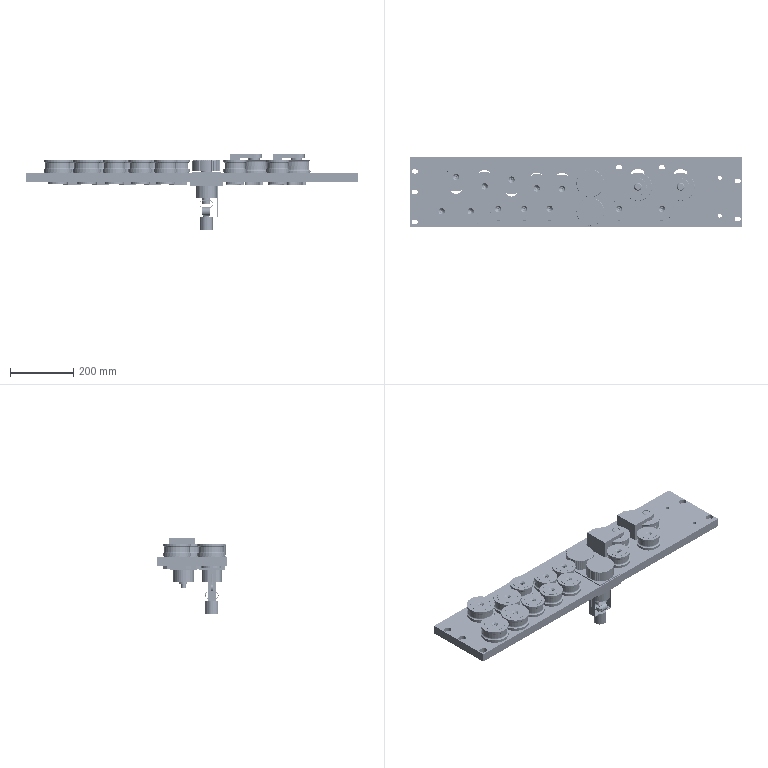Assembly | SolidWorks | mm | 86 component files | 278 solids | 5962 faces | box 1050 x 220 x 237.51 mm | volume 10326215 mm3 | cylinder 1953 | plane 1541 | sphere 1504 | cone 570 | torus 394 | commonest cylinder face diameters 34.9 x282 37.1 x282 8.5 x124 88 x88 86 x86 11 x74 45 x67 55 x64
Bill of materials:
12ACoupling | 1 |  | Two thin-walled stadium (obround) loops arranged at right angles to each other and touching at one point. Each loop holds a cylindrical collar with a central through bore and a small radial hole with a recessed socket feature on its side.
12AEncoder | 1 |  | Solid cylindrical body. A smaller coaxial cylindrical boss sits on one end face, and a thin shaft sticks out of the boss. Three small holes are spaced evenly around the end face.
12AEncoderBracket | 1 | Q235 | Formed sheet-style U-shaped bracket. The flat base has a circular lobe with a large central hole and three small holes around it. Two vertical side walls each have a long vertical slot. Each wall ends in an outward-bent tab with one hole and rounded corners.
12A6005RZBearing | 6 |  | Flat annular ring with a plain cylindrical outer surface and a smooth through-bore. The end face has concentric bands: an outer rim, a wide middle annular face, and a narrow inner ring band near the bore, separated by shallow circular grooves/steps. Overall it looks like a shielded deep-groove ball bearing (outer ring, shield, inner ring), but this is only inferred from shape.
12A6006RZBearing | 2 |  | Annular ring with a rectangular cross-section and rounded edges. The face has shallow concentric step or groove rings between the inner and outer diameters.
12AEncoderAxis | 2 |  | Axisymmetric pin with a large cylindrical head ridged around its edge. Below the head is a stepped shaft that gets narrower in stages. Near the lower end there is a narrow groove and a small end pilot.
12AEncoderAxisFrontBaffle | 2 | Q235 | Thin square plate with a central round through hole. Below the plate is a slightly smaller block with a rounded-square outline.
12AEncoderAxisRearBaffle | 2 | Q235 | Flanged cylindrical housing. A rectangular flange plate has four larger corner holes, two small holes on the short-side centerlines, and a large central through bore. A cylindrical body extends below the plate and a short stepped spigot rises above it.
12AFlatSlotLargeStraighteningWheel | 4 | GCr15 | Spool-shaped wheel with two end flanges and a concave circumferential groove between them. It has a central through bore and a shallow annular groove on the end face.
12ALargeStraighteningWheelAxis | 4 | Q235 | Stepped axisymmetric part. A wide thin flange disc has raised concentric step rings on top. An upper cylinder with a small central hole rises from it, and a larger lower cylinder with chamfered ends sits below.
12ALargeStraighteningWheelCover | 4 | 45 | Thin flat disc with a central countersunk through hole. A shallow stepped boss with a chamfered edge sits on the underside.
12AFixedLargeStraighteningWheelBaffle | 7 | Q235 | Plain flat circular disc with a small central through hole.
12AFlatSlotSmallStraighteningWheel | 8 | GCr15 | Spool-shaped wheel with two end flanges and a concave radiused groove between them. It has a central through bore and an annular groove on the end face. It is proportionally taller, with a relatively larger bore than the similar spool part.
12ASmallStraighteningWheelAxis | 8 | 45 | Stepped, mostly revolved body: a small cylindrical boss on top with a small central hole, a raised annular step, a thin wide flange, and a larger lower cylindrical body with one flat side.
12ASmallStraighteningWheelCover | 8 | 45 | Thin flat circular disc with a central countersunk through hole, plus a shallow stepped boss on the underside.
12A6006DeepGrooveBallBearing | 4 | GCr4 | Ball-bearing-like geometry: concentric outer and inner rings with a ring of spherical balls between them. No shield or cage is visible.
12AInnerSideWheel | 2 | Cr12MoV | Short annular ring with a central through bore and a thin outward flange at its base, joined to the ring wall by a fillet.
12AInnerSideWheelAxis | 2 | 45 | Stepped, mostly revolved body: a solid small cylindrical boss on top, a raised annular step, two flange tiers, and a larger lower cylindrical body with one flat side.
12AOuterSideWheel | 2 | Cr12MoV | Flanged cylindrical sleeve: a short tube with a thin outward flange at one end and a stepped internal bore.
12AOuterSideWheelPlate | 2 | Q235 | Flat plate of uniform thickness: two straight edges meeting at a corner, an angled edge, and a rounded lobe at one end with a single round through hole. There is a small rectangular notch in one edge.
12AOuterSideWheelSeat | 2 | Q235 | T-shaped block: a rectangular upper block with a narrow raised rib running along its top, and a narrower lower extension with a rounded end.
12AOuterSideWheelSmallAxis | 2 | 45 | Solid stepped cylindrical plug: a chamfered top cylinder, a wider collar or flange, and a main cylindrical body with a circumferential groove near the lower end.
12ASlidingPlateWheelCover | 4 | Q235 | Flat rectangular plate with rounded corners, a concave circular-arc cutout along one short edge, and two round through holes in line on the centerline.
12ASlidingStraighteningWheelRetainingPlate | 5 | Q235 | Flat rectangular plate with all four corners chamfered (elongated octagon outline) and two round through holes on the centerline.
12AStraighteningPlate | 1 | Q235 | Long, thin rectangular panel plate with many cutouts in two rows: rounded or D-shaped oblong openings, two square openings, two narrow slots, and small holes and slots near both ends.
Mates:
1. coincident | 12AStraighteningPlate-1 face at (-449.402, 230.038, 14.25) dir (0, 0, 1) | 12AFixedFlatGrooveLargeWheel-EngravingAndMillingAxis-2/12ALargeStraighteningWheelAxis-1 face at (-257.402, 101.538, 14.25) dir (0, 0, -1)
2. coincident | 12AStraighteningPlate-1 face at (-449.402, 230.038, 14.25) dir (0, 0, 1) | 12AFixedFlatGrooveLargeWheel-EngravingAndMillingAxis-3/12ALargeStraighteningWheelAxis-1 face at (-349.402, 101.538, 14.25) dir (0, 0, -1)
3. coincident | 12AStraighteningPlate-1 face at (-363.544, 76.538, -14.25) dir (0, -1, 0) | 12AFixedFlatGrooveLargeWheel-EngravingAndMillingAxis-3/12ALargeStraighteningWheelAxis-1 face at (-335.259, 76.538, 42.973) dir (0, 1, 0)
4. concentric | 12AStraighteningPlate-1 face at (-349.402, 59.038, -14.25) dir (0, 0, 1) r 22.5 | 12AFixedFlatGrooveLargeWheel-EngravingAndMillingAxis-3/12ALargeStraighteningWheelAxis-1 face at (-349.402, 59.038, -14.25) dir (0, 0, -1) r 22.5
5. coincident | 12AStraighteningPlate-1 face at (-271.544, 76.538, -14.25) dir (0, -1, 0) | 12AFixedFlatGrooveLargeWheel-EngravingAndMillingAxis-2/12ALargeStraighteningWheelAxis-1 face at (-243.259, 76.538, 42.973) dir (0, 1, 0)
6. concentric | 12AStraighteningPlate-1 face at (-257.402, 59.038, -14.25) dir (0, 0, 1) r 22.5 | 12AFixedFlatGrooveLargeWheel-EngravingAndMillingAxis-2/12ALargeStraighteningWheelAxis-1 face at (-257.402, 59.038, -14.25) dir (0, 0, -1) r 22.5
7. coincident | 12AStraighteningPlate-1 face at (-449.402, 230.038, 14.25) dir (0, 0, 1) | 12AFlatGrooveSmallWheel-MillingAxis-5/12ASmallStraighteningWheelAxis-1 face at (346.598, 101.038, 14.25) dir (0, 0, -1)
8. coincident | 12AStraighteningPlate-1 face at (-449.402, 230.038, 14.25) dir (0, 0, 1) | 12AFlatGrooveSmallWheel-MillingAxis-4/12ASmallStraighteningWheelAxis-1 face at (211.598, 101.038, 14.25) dir (0, 0, -1)
9. coincident | 12AStraighteningPlate-1 face at (-449.402, 230.038, 14.25) dir (0, 0, 1) | 12AFlatGrooveSmallWheel-MillingAxis-3/12ASmallStraighteningWheelAxis-1 face at (-8.402, 101.038, 14.25) dir (0, 0, -1)
10. coincident | 12AStraighteningPlate-1 face at (-449.402, 230.038, 14.25) dir (0, 0, 1) | 12AFlatGrooveSmallWheel-MillingAxis-1/12ASmallStraighteningWheelAxis-1 face at (-170.402, 101.038, 14.25) dir (0, 0, -1)
11. coincident | 12AStraighteningPlate-1 face at (-449.402, 230.038, 14.25) dir (0, 0, 1) | 12AFlatGrooveSmallWheel-MillingAxis-2/12ASmallStraighteningWheelAxis-1 face at (-88.402, 101.038, 14.25) dir (0, 0, -1)
12. coincident | 12AStraighteningPlate-1 face at (-184.544, 84.038, -14.25) dir (0, -1, 0) | 12AFlatGrooveSmallWheel-MillingAxis-1/12ASmallStraighteningWheelAxis-1 face at (-156.259, 84.038, 42.973) dir (0, 1, 0)
13. concentric | 12AStraighteningPlate-1 face at (-170.402, 66.538, -14.25) dir (0, 0, 1) r 22.5 | 12AFlatGrooveSmallWheel-MillingAxis-1/12ASmallStraighteningWheelAxis-1 face at (-170.402, 66.538, -14.25) dir (0, 0, -1) r 22.5
14. coincident | 12AStraighteningPlate-1 face at (-102.544, 84.038, -14.25) dir (0, -1, 0) | 12AFlatGrooveSmallWheel-MillingAxis-2/12ASmallStraighteningWheelAxis-1 face at (-74.259, 84.038, 42.973) dir (0, 1, 0)
15. concentric | 12AStraighteningPlate-1 face at (-88.402, 66.538, -14.25) dir (0, 0, 1) r 22.5 | 12AFlatGrooveSmallWheel-MillingAxis-2/12ASmallStraighteningWheelAxis-1 face at (-88.402, 66.538, -14.25) dir (0, 0, -1) r 22.5
16. coincident | 12AStraighteningPlate-1 face at (-22.544, 84.038, -14.25) dir (0, -1, 0) | 12AFlatGrooveSmallWheel-MillingAxis-3/12ASmallStraighteningWheelAxis-1 face at (5.741, 84.038, 42.973) dir (0, 1, 0)
17. concentric | 12AStraighteningPlate-1 face at (-8.402, 66.538, -14.25) dir (0, 0, 1) r 22.5 | 12AFlatGrooveSmallWheel-MillingAxis-3/12ASmallStraighteningWheelAxis-1 face at (-8.402, 66.538, -14.25) dir (0, 0, -1) r 22.5
18. coincident | 12AStraighteningPlate-1 face at (197.456, 49.038, -14.25) dir (0, 1, 0) | 12AFlatGrooveSmallWheel-MillingAxis-4/12ASmallStraighteningWheelAxis-1 face at (225.741, 49.038, 42.973) dir (0, -1, 0)
19. concentric | 12AStraighteningPlate-1 face at (211.598, 66.538, -14.25) dir (0, 0, 1) r 22.5 | 12AFlatGrooveSmallWheel-MillingAxis-4/12ASmallStraighteningWheelAxis-1 face at (211.598, 66.538, -14.25) dir (0, 0, -1) r 22.5
20. coincident | 12AStraighteningPlate-1 face at (332.456, 84.038, -14.25) dir (0, -1, 0) | 12AFlatGrooveSmallWheel-MillingAxis-5/12ASmallStraighteningWheelAxis-1 face at (360.741, 84.038, 42.973) dir (0, 1, 0)
21. concentric | 12AStraighteningPlate-1 face at (346.598, 66.538, -14.25) dir (0, 0, 1) r 22.5 | 12AFlatGrooveSmallWheel-MillingAxis-5/12ASmallStraighteningWheelAxis-1 face at (346.598, 66.538, -14.25) dir (0, 0, -1) r 22.5
22. coincident | 12AStraighteningPlate-1 face at (-449.402, 230.038, 14.25) dir (0, 0, 1) | 12ASlidingFlatGrooveLargeWheel-MillingAxis-3/12ALargeStraighteningWheelAxis-1 face at (-260.902, 167.538, 14.25) dir (0, 0, -1)
23. coincident | 12AStraighteningPlate-1 face at (-285.902, 181.68, -14.25) dir (-1, 0, 0) | 12ASlidingFlatGrooveLargeWheel-MillingAxis-3/12ALargeStraighteningWheelAxis-1 face at (-285.902, 153.396, 42.973) dir (1, 0, 0)
24. concentric | 12AStraighteningPlate-1 face at (-303.402, 167.538, -14.25) dir (0, 0, 1) r 22.5 | 12ASlidingFlatGrooveLargeWheel-MillingAxis-3/12ALargeStraighteningWheelAxis-1 face at (-303.402, 167.538, -14.25) dir (0, 0, -1) r 22.5
25. coincident | 12AStraighteningPlate-1 face at (-230.902, 181.68, -14.25) dir (1, 0, 0) | 12ASlidingFlatGrooveLargeWheel-MillingAxis-2/12ALargeStraighteningWheelAxis-1 face at (-230.902, 123.586, 42.973) dir (-1, 0, 0)
26. coincident | 12AStraighteningPlate-1 face at (-449.402, 230.038, 14.25) dir (0, 0, 1) | 12ASlidingFlatGrooveLargeWheel-MillingAxis-2/12ALargeStraighteningWheelAxis-1 face at (-170.902, 137.728, 14.25) dir (0, 0, -1)
27. coincident | 12AStraighteningPlate-1 face at (-449.402, 230.038, 14.25) dir (0, 0, 1) | 12ASlidingFlatGrooveSmallWheel-MillingAxis-1/12ASmallStraighteningWheelAxis-1 face at (66.098, 130.148, 14.25) dir (0, 0, -1)
28. coincident | 12AStraighteningPlate-1 face at (-449.402, 230.038, 14.25) dir (0, 0, 1) | 12ASlidingFlatGrooveSmallWheel-MillingAxis-2/12ASmallStraighteningWheelAxis-1 face at (-13.902, 131.343, 14.25) dir (0, 0, -1)
29. coincident | 12AStraighteningPlate-1 face at (-449.402, 230.038, 14.25) dir (0, 0, 1) | 12ASlidingFlatGrooveSmallWheel-MillingAxis-3/12ASmallStraighteningWheelAxis-1 face at (-93.902, 159.038, 14.25) dir (0, 0, -1)
30. coincident | 12AStraighteningPlate-1 face at (49.098, 173.18, -14.25) dir (-1, 0, 0) | 12ASlidingFlatGrooveSmallWheel-MillingAxis-1/12ASmallStraighteningWheelAxis-1 face at (49.098, 116.006, 42.973) dir (1, 0, 0)
31. coincident | 12AStraighteningPlate-1 face at (-30.902, 173.18, -14.25) dir (-1, 0, 0) | 12ASlidingFlatGrooveSmallWheel-MillingAxis-2/12ASmallStraighteningWheelAxis-1 face at (-30.902, 117.201, 42.973) dir (1, 0, 0)
32. coincident | 12AStraighteningPlate-1 face at (-110.902, 173.18, -14.25) dir (-1, 0, 0) | 12ASlidingFlatGrooveSmallWheel-MillingAxis-3/12ASmallStraighteningWheelAxis-1 face at (-110.902, 144.896, 42.973) dir (1, 0, 0)
33. coincident | 12AStraighteningPlate-1 face at (-449.402, 230.038, 14.25) dir (0, 0, 1) | 12AInnerSideWheel-EngravingAndMillingAxis-1/12AInnerSideWheelAxis-2 face at (271.598, 173.038, 14.25) dir (0, 0, -1)
34. coincident | 12AInnerSideWheel-EngravingAndMillingAxis-1/12AInnerSideWheelAxis-2 face at (292.098, 167.483, 77.467) dir (1, 0, 0) | 12AStraighteningPlate-1 face at (292.098, 183.03, -14.25) dir (-1, 0, 0)
35. concentric | 12AStraighteningPlate-1 face at (271.598, 137.038, -14.25) dir (0, 0, 1) r 26 | 12AInnerSideWheel-EngravingAndMillingAxis-1/12AInnerSideWheelAxis-2 face at (271.598, 137.038, -14.25) dir (0, 0, -1) r 26
36. coincident | 12AStraighteningPlate-1 face at (-449.402, 230.038, 14.25) dir (0, 0, 1) | 12AOuterSideWheel-EngravingAndMillingAxis-1/12AOuterSideWheelSeat-1 face at (226.598, 111.538, 14.25) dir (0, 0, -1)
37. coincident | 12AStraighteningPlate-1 face at (202.598, 197.538, -14.25) dir (1, 0, 0) | 12AOuterSideWheel-EngravingAndMillingAxis-1/12AOuterSideWheelSeat-1 face at (202.598, 126.538, -14.25) dir (-1, 0, 0)
38. concentric | 12AStraighteningPlate-1 face at (211.598, 126.538, -14.25) dir (0, 0, 1) r 9 | 12AOuterSideWheel-EngravingAndMillingAxis-1/12AOuterSideWheelSeat-1 face at (211.598, 126.538, -14.25) dir (0, 0, 1) r 9
39. coincident | 12AStraighteningPlate-1 face at (-449.402, 230.038, 14.25) dir (0, 0, 1) | 12AInnerSideWheel-EngravingAndMillingAxis-2/12AInnerSideWheelAxis-2 face at (406.598, 173.038, 14.25) dir (0, 0, -1)
40. concentric | 12AStraighteningPlate-1 face at (406.598, 137.038, -14.25) dir (0, 0, 1) r 26 | 12AInnerSideWheel-EngravingAndMillingAxis-2/12AInnerSideWheelAxis-2 face at (406.598, 137.038, -14.25) dir (0, 0, -1) r 26
41. coincident | 12AStraighteningPlate-1 face at (355.598, 197.538, -14.25) dir (-1, 0, 0) | 12AOuterSideWheel-EngravingAndMillingAxis-2/12AOuterSideWheelSeat-1 face at (355.598, 126.538, -14.25) dir (1, 0, 0)
42. concentric | 12AStraighteningPlate-1 face at (346.598, 126.538, -14.25) dir (0, 0, 1) r 9 | 12AOuterSideWheel-EngravingAndMillingAxis-2/12AOuterSideWheelSeat-1 face at (346.598, 126.538, -14.25) dir (0, 0, 1) r 9
43. coincident | 12AStraighteningPlate-1 face at (-449.402, 230.038, 14.25) dir (0, 0, 1) | 12AOuterSideWheel-EngravingAndMillingAxis-2/12AOuterSideWheelSeat-1 face at (361.598, 111.538, 14.25) dir (0, 0, -1)
44. coincident | 12AStraighteningPlate-1 face at (-449.402, 230.038, -14.25) dir (0, 0, -1) | 12AFixedLargeStraighteningWheelBaffle-12 face at (-349.402, 59.038, -14.25) dir (0, 0, 1)
45. concentric | 12AFixedFlatGrooveLargeWheel-EngravingAndMillingAxis-3/12ALargeStraighteningWheelAxis-1 face at (-349.402, 59.038, -14.25) dir (0, 0, -1) r 4.25 | 12AFixedLargeStraighteningWheelBaffle-12 face at (-349.402, 59.038, -20.25) dir (0, 0, 1) r 5.5
46. coincident | 12AStraighteningPlate-1 face at (-449.402, 230.038, -14.25) dir (0, 0, -1) | 12AFixedLargeStraighteningWheelBaffle-11 face at (-257.402, 59.038, -14.25) dir (0, 0, 1)
47. concentric | 12AFixedFlatGrooveLargeWheel-EngravingAndMillingAxis-2/12ALargeStraighteningWheelAxis-1 face at (-257.402, 59.038, -14.25) dir (0, 0, -1) r 4.25 | 12AFixedLargeStraighteningWheelBaffle-11 face at (-257.402, 59.038, -20.25) dir (0, 0, 1) r 5.5
48. concentric | 12AFlatGrooveSmallWheel-MillingAxis-1/12ASmallStraighteningWheelAxis-1 face at (-170.402, 66.538, -14.25) dir (0, 0, -1) r 4.25 | 12AFixedLargeStraighteningWheelBaffle-2 face at (-170.402, 66.538, -20.25) dir (0, 0, 1) r 5.5
49. coincident | 12AStraighteningPlate-1 face at (-449.402, 230.038, -14.25) dir (0, 0, -1) | 12AFixedLargeStraighteningWheelBaffle-2 face at (-170.402, 66.538, -14.25) dir (0, 0, 1)
50. coincident | 12AStraighteningPlate-1 face at (-449.402, 230.038, -14.25) dir (0, 0, -1) | 12AFixedLargeStraighteningWheelBaffle-3 face at (-88.402, 66.538, -14.25) dir (0, 0, 1)
51. concentric | 12AFlatGrooveSmallWheel-MillingAxis-2/12ASmallStraighteningWheelAxis-1 face at (-88.402, 66.538, -14.25) dir (0, 0, -1) r 4.25 | 12AFixedLargeStraighteningWheelBaffle-3 face at (-88.402, 66.538, -14.25) dir (0, 0, -1) r 5.5
52. concentric | 12AFlatGrooveSmallWheel-MillingAxis-3/12ASmallStraighteningWheelAxis-1 face at (-8.402, 66.538, -14.25) dir (0, 0, -1) r 4.25 | 12AFixedLargeStraighteningWheelBaffle-8 face at (-8.402, 66.538, -20.25) dir (0, 0, 1) r 5.5
53. coincident | 12AStraighteningPlate-1 face at (-449.402, 230.038, -14.25) dir (0, 0, -1) | 12AFixedLargeStraighteningWheelBaffle-8 face at (-8.402, 66.538, -14.25) dir (0, 0, 1)
54. concentric | 12AFlatGrooveSmallWheel-MillingAxis-4/12ASmallStraighteningWheelAxis-1 face at (211.598, 66.538, -14.25) dir (0, 0, -1) r 4.25 | 12AFixedLargeStraighteningWheelBaffle-6 face at (211.598, 66.538, -20.25) dir (0, 0, 1) r 5.5
55. coincident | 12AStraighteningPlate-1 face at (-449.402, 230.038, -14.25) dir (0, 0, -1) | 12AFixedLargeStraighteningWheelBaffle-6 face at (211.598, 66.538, -14.25) dir (0, 0, 1)
56. coincident | 12AFlatGrooveSmallWheel-MillingAxis-5/12ASmallStraighteningWheelAxis-1 face at (346.598, 88.038, -14.25) dir (0, 0, -1) | 12AFixedLargeStraighteningWheelBaffle-5 face at (346.598, 66.538, -14.25) dir (0, 0, 1)
57. concentric | 12AFlatGrooveSmallWheel-MillingAxis-5/12ASmallStraighteningWheelAxis-1 face at (346.598, 66.538, -14.25) dir (0, 0, -1) r 4.25 | 12AFixedLargeStraighteningWheelBaffle-5 face at (346.598, 66.538, -20.25) dir (0, 0, 1) r 5.5
58. concentric | 12ASlidingFlatGrooveLargeWheel-MillingAxis-3/12ALargeStraighteningWheelAxis-1 face at (-303.402, 152.538, -14.25) dir (0, 0, -1) r 4.25 | 12ASlidingStraighteningWheelRetainingPlate-5 edge at (-303.402, 152.538, -14.25) dir (0, 0, 1) r 5.5
59. concentric | 12ASlidingFlatGrooveLargeWheel-MillingAxis-3/12ALargeStraighteningWheelAxis-1 face at (-303.402, 182.538, -14.25) dir (0, 0, -1) r 4.25 | 12ASlidingStraighteningWheelRetainingPlate-5 face at (-303.402, 182.538, -14.25) dir (0, 0, 1) r 5.5
60. coincident | 12ASlidingFlatGrooveLargeWheel-MillingAxis-3/12ALargeStraighteningWheelAxis-1 face at (-281.902, 167.538, -14.25) dir (0, 0, -1) | 12ASlidingStraighteningWheelRetainingPlate-5 face at (-303.402, 167.538, -14.25) dir (0, 0, 1)
61. coincident | 12ASlidingFlatGrooveLargeWheel-MillingAxis-2/12ALargeStraighteningWheelAxis-1 face at (-191.902, 137.728, -14.25) dir (0, 0, -1) | 12ASlidingStraighteningWheelRetainingPlate-3 face at (-128.402, 159.038, -14.25) dir (0, 0, 1)
62. concentric | 12ASlidingFlatGrooveLargeWheel-MillingAxis-2/12ALargeStraighteningWheelAxis-1 face at (-213.402, 122.728, -14.25) dir (0, 0, -1) r 4.25 | 12ASlidingStraighteningWheelRetainingPlate-2 face at (-213.402, 122.728, -14.25) dir (0, 0, 1) r 5.5
63. concentric | 12ASlidingFlatGrooveLargeWheel-MillingAxis-2/12ALargeStraighteningWheelAxis-1 face at (-213.402, 152.728, -14.25) dir (0, 0, -1) r 4.25 | 12ASlidingStraighteningWheelRetainingPlate-2 face at (-213.402, 152.728, -14.25) dir (0, 0, 1) r 5.5
64. coincident | 12ASlidingFlatGrooveSmallWheel-MillingAxis-3/12ASmallStraighteningWheelAxis-1 face at (-106.902, 159.038, -14.25) dir (0, 0, -1) | 12ASlidingStraighteningWheelRetainingPlate-3 face at (-128.402, 159.038, -14.25) dir (0, 0, 1)
65. concentric | 12ASlidingFlatGrooveSmallWheel-MillingAxis-3/12ASmallStraighteningWheelAxis-1 face at (-128.402, 144.038, -14.25) dir (0, 0, -1) r 4.25 | 12ASlidingStraighteningWheelRetainingPlate-3 face at (-128.402, 144.038, -14.25) dir (0, 0, 1) r 5.5
66. concentric | 12ASlidingFlatGrooveSmallWheel-MillingAxis-3/12ASmallStraighteningWheelAxis-1 face at (-128.402, 174.038, -14.25) dir (0, 0, -1) r 4.25 | 12ASlidingStraighteningWheelRetainingPlate-3 face at (-128.402, 174.038, -14.25) dir (0, 0, 1) r 5.5
67. concentric | 12ASlidingFlatGrooveSmallWheel-MillingAxis-2/12ASmallStraighteningWheelAxis-1 face at (-48.402, 116.343, -14.25) dir (0, 0, -1) r 4.25 | 12ASlidingStraighteningWheelRetainingPlate-4 face at (-48.402, 116.343, -14.25) dir (0, 0, 1) r 5.5
68. concentric | 12ASlidingFlatGrooveSmallWheel-MillingAxis-2/12ASmallStraighteningWheelAxis-1 face at (-48.402, 146.343, -14.25) dir (0, 0, -1) r 4.25 | 12ASlidingStraighteningWheelRetainingPlate-4 edge at (-48.402, 146.343, -24.25) dir (0, 0, -1) r 5.5
69. coincident | 12AStraighteningPlate-1 face at (-449.402, 230.038, -14.25) dir (0, 0, -1) | 12ASlidingStraighteningWheelRetainingPlate-4 face at (-48.402, 131.343, -14.25) dir (0, 0, 1)
70. coincident | 12ASlidingFlatGrooveSmallWheel-MillingAxis-1/12ASmallStraighteningWheelAxis-1 face at (53.098, 130.148, -14.25) dir (0, 0, -1) | 12ASlidingStraighteningWheelRetainingPlate-6 face at (31.598, 130.148, -14.25) dir (0, 0, 1)
71. concentric | 12ASlidingFlatGrooveSmallWheel-MillingAxis-1/12ASmallStraighteningWheelAxis-1 face at (31.598, 115.148, -14.25) dir (0, 0, -1) r 4.25 | 12ASlidingStraighteningWheelRetainingPlate-6 face at (31.598, 115.148, -14.25) dir (0, 0, 1) r 5.5
72. concentric | 12ASlidingFlatGrooveSmallWheel-MillingAxis-1/12ASmallStraighteningWheelAxis-1 face at (31.598, 145.148, -14.25) dir (0, 0, -1) r 4.25 | 12ASlidingStraighteningWheelRetainingPlate-6 face at (31.598, 145.148, -14.25) dir (0, 0, 1) r 5.5
73. coincident | 12AStraighteningPlate-1 face at (-449.402, 230.038, -14.25) dir (0, 0, -1) | 12ASlidingPlateWheelCover-1 face at (211.598, 136.538, -14.25) dir (0, 0, 1)
74. coincident | 12AStraighteningPlate-1 face at (-449.402, 230.038, -14.25) dir (0, 0, -1) | 12ASlidingPlateWheelCover-2 face at (271.598, 129.538, -14.25) dir (0, 0, 1)
75. coincident | 12AStraighteningPlate-1 face at (-449.402, 230.038, -14.25) dir (0, 0, -1) | 12ASlidingPlateWheelCover-3 face at (346.598, 136.538, -14.25) dir (0, 0, 1)
76. coincident | 12AStraighteningPlate-1 face at (-449.402, 230.038, -14.25) dir (0, 0, -1) | 12ASlidingPlateWheelCover-4 face at (406.598, 129.538, -14.25) dir (0, 0, 1)
77. concentric | 12AInnerSideWheel-EngravingAndMillingAxis-2/12AInnerSideWheelAxis-2 face at (406.598, 119.538, -14.25) dir (0, 0, -1) r 5.1 | 12ASlidingPlateWheelCover-4 face at (406.598, 119.538, -14.25) dir (0, 0, -1) r 6.5
78. concentric | 12AInnerSideWheel-EngravingAndMillingAxis-2/12AInnerSideWheelAxis-2 face at (406.598, 139.538, -14.25) dir (0, 0, -1) r 5.1 | 12ASlidingPlateWheelCover-4 face at (406.598, 139.538, -14.25) dir (0, 0, -1) r 6.5
79. concentric | 12AOuterSideWheel-EngravingAndMillingAxis-2/12AOuterSideWheelSeat-1 face at (346.598, 126.538, -14.25) dir (0, 0, -1) r 4.25 | 12ASlidingPlateWheelCover-3 face at (346.598, 126.538, -14.25) dir (0, 0, -1) r 6.5
80. concentric | 12AOuterSideWheel-EngravingAndMillingAxis-2/12AOuterSideWheelSeat-1 face at (346.598, 146.538, -14.25) dir (0, 0, -1) r 4.25 | 12ASlidingPlateWheelCover-3 face at (346.598, 146.538, -14.25) dir (0, 0, -1) r 6.5
81. concentric | 12AInnerSideWheel-EngravingAndMillingAxis-1/12AInnerSideWheelAxis-2 face at (271.598, 119.538, -14.25) dir (0, 0, -1) r 5.1 | 12ASlidingPlateWheelCover-2 face at (271.598, 119.538, -14.25) dir (0, 0, -1) r 6.5
82. concentric | 12AInnerSideWheel-EngravingAndMillingAxis-1/12AInnerSideWheelAxis-2 face at (271.598, 139.538, -14.25) dir (0, 0, -1) r 5.1 | 12ASlidingPlateWheelCover-2 face at (271.598, 139.538, -14.25) dir (0, 0, -1) r 6.5
83. concentric | 12AOuterSideWheel-EngravingAndMillingAxis-1/12AOuterSideWheelSeat-1 face at (211.598, 126.538, -14.25) dir (0, 0, -1) r 4.25 | 12ASlidingPlateWheelCover-1 face at (211.598, 126.538, -14.25) dir (0, 0, -1) r 6.5
84. concentric | 12AOuterSideWheel-EngravingAndMillingAxis-1/12AOuterSideWheelSeat-1 face at (211.598, 146.538, -14.25) dir (0, 0, -1) r 4.25 | 12ASlidingPlateWheelCover-1 face at (211.598, 146.538, -14.25) dir (0, 0, -1) r 6.5
85. coincident | 12AStraighteningPlate-1 face at (164.894, 180.671, -245.75) dir (-1, 0, 0) | 12AEncoderWheel-1/12AEncoderAxisFrontBaffle-1 face at (164.894, 172.181, -14.25) dir (1, 0, 0)
86. coincident | 12AStraighteningPlate-1 face at (-449.402, 230.038, 14.25) dir (0, 0, 1) | 12AEncoderWheel-1/12AEncoderAxisFrontBaffle-1 face at (120.894, 147.181, 14.25) dir (0, 0, -1)
87. coincident | 12AStraighteningPlate-1 face at (76.894, 82.671, -245.75) dir (1, 0, 0) | 12AEncoderWheel-2/12AEncoderAxisFrontBaffle-1 face at (76.894, 82.671, -14.25) dir (-1, 0, 0)
88. coincident | 12AStraighteningPlate-1 face at (86.894, 92.671, -245.75) dir (0, -1, 0) | 12AEncoderWheel-2/12AEncoderAxisFrontBaffle-1 face at (86.894, 92.671, -14.25) dir (0, 1, 0)
89. coincident | 12AStraighteningPlate-1 face at (-449.402, 230.038, 14.25) dir (0, 0, 1) | 12AEncoderWheel-2/12AEncoderAxisFrontBaffle-1 face at (120.894, 57.671, 14.25) dir (0, 0, -1)
90. concentric | 12AEncoderWheel-2/12AEncoderAxisRearBaffle-1 face at (168.394, 57.671, -26.25) dir (0, 0, -1) r 2.5 | 12AEncoderBracket-1 face at (168.394, 57.671, -26.25) dir (0, 0, 1) r 3.5
91. concentric | 12AEncoderWheel-2/12AEncoderAxisRearBaffle-1 face at (73.394, 57.671, -26.25) dir (0, 0, -1) r 2.5 | 12AEncoderBracket-1 face at (73.394, 57.671, -26.25) dir (0, 0, 1) r 3.5
92. coincident | 12AEncoderWheel-2/12AEncoderAxisRearBaffle-1 face at (120.894, 57.671, -26.25) dir (0, 0, -1) | 12AEncoderBracket-1 face at (120.894, 57.671, -26.25) dir (0, 0, 1)
93. concentric | 12AEncoderWheel-2/12AEncoderAxis-1 face at (120.894, 57.671, -85.75) dir (0, 0, 1) r 7.5 | 12ACoupling-1 face at (120.894, 57.671, -83.975) dir (0, 0, -1) r 7.5
94. concentric | 12AEncoderBracket-1 face at (120.894, 57.671, -116.26) dir (0, 0, -1) r 10.5 | 12AEncoder-1 face at (120.894, 57.671, -165.26) dir (0, 0, -1) r 20
95. concentric | 12AEncoderBracket-1 edge at (107.903, 65.171, -126.26) dir (0, 0, -1) r 2 | 12AEncoder-1 face at (107.903, 65.171, -126.26) dir (0, 0, 1) r 1.25
96. concentric | 12AEncoderBracket-1 face at (120.894, 57.671, -116.26) dir (0, 0, -1) r 10.5 | 12AEncoder-1 face at (120.894, 57.671, -165.26) dir (0, 0, -1) r 10
97. coincident | 12AEncoderBracket-1 face at (120.894, 57.671, -126.26) dir (0, 0, -1) | 12AEncoder-1 face at (112.234, 62.671, -126.26) dir (0, 0, 1)
98. concentric | 12AStraighteningPlate-1 face at (-128.402, 159.038, -14.25) dir (0, 0, 1) r 22.5 | 12ASlidingFlatGrooveSmallWheel-MillingAxis-3/12ASmallStraighteningWheelAxis-1 face at (-128.402, 159.038, -14.25) dir (0, 0, -1) r 22.5
99. coincident | 12ASlidingFlatGrooveLargeWheel-MillingAxis-2/12ALargeStraighteningWheelAxis-1 face at (-191.902, 137.728, -14.25) dir (0, 0, -1) | 12ASlidingStraighteningWheelRetainingPlate-2 face at (-213.402, 137.728, -14.25) dir (0, 0, 1)
100. concentric | 12AEncoderAxis-1 face at (76.773, 3.026, 0.00888) dir (0, -1, 0) r 15 | 12AEncoderAxisFrontBaffle-1 face at (76.773, -30.474, 0.00888) dir (0, 1, 0) r 27.5
101. concentric | 12AEncoderAxis-1 face at (76.773, 48.026, 0.00888) dir (0, -1, 0) r 12.5 | 12AEncoderAxisRearBaffle-1 face at (76.773, 44.026, 0.00888) dir (0, -1, 0) r 32.5
102. concentric | 12AEncoderAxis-1 face at (76.773, 3.026, 0.00888) dir (0, -1, 0) r 15 | 12A6006RZBearing-1 face at (76.773, -5030.474, 0.00888) dir (0, 1, 0) r 27.5
103. coincident | 12AEncoderAxisFrontBaffle-1 face at (85.558, -8.474, 41.286) dir (0, 1, 0) | 12AEncoderAxisRearBaffle-1 face at (76.773, -8.474, 0.00888) dir (0, -1, 0)
104. parallel | 12AEncoderAxisFrontBaffle-1 face at (93.03, -8.474, 47.933) dir (0.7471, 0, 0.6647) | 12AEncoderAxisRearBaffle-1 face at (88.413, 3.526, 65.91) dir (0.7471, 0, 0.6647)
105. concentric | 12A6005RZBearing-1 face at (76.773, 12.526, 0.00888) dir (0, 1, 0) r 23.5 | 12A6005RZBearing-2 face at (76.773, 24.526, 0.00888) dir (0, 1, 0) r 23.5
106. concentric | 12A6005RZBearing-2 face at (76.773, 24.526, 0.00888) dir (0, 1, 0) r 23.5 | 12A6005RZBearing-4 face at (76.773, 36.526, 0.00888) dir (0, 1, 0) r 23.5
107. coincident | 12A6005RZBearing-2 face at (99.673, 27.026, 0.00888) dir (0, 1, 0) | 12A6005RZBearing-4 face at (99.637, 27.026, -1.271) dir (0, -1, 0)
108. coincident | 12A6005RZBearing-1 face at (99.65, 15.026, 1.033) dir (0, 1, 0) | 12A6005RZBearing-2 face at (99.673, 15.026, 0.00888) dir (0, -1, 0)
109. concentric | 12AEncoderAxisRearBaffle-1 face at (76.773, 44.026, 0.00888) dir (0, -1, 0) r 32.5 | 12A6005RZBearing-4 face at (76.773, 36.526, 0.00888) dir (0, 1, 0) r 23.5
110. parallel | 12AEncoderAxisFrontBaffle-1 face at (76.773, -17.474, 0.00888) dir (0, 1, 0) | 12A6006RZBearing-1 face at (103.245, -17.474, -1.204) dir (0, 1, 0)
111. distance | 12AEncoderAxisFrontBaffle-1 face at (76.773, -40.474, 0.00888) dir (0, -1, 0) | 12AEncoderAxis-1 face at (76.773, -41.474, 0.00888) dir (0, 1, 0)
112. coincident | 12AEncoderAxis-1 face at (76.773, 3.026, 0.00888) dir (0, 1, 0) | 12A6005RZBearing-1 face at (91.702, 3.026, 0.6771) dir (0, -1, 0)
113. concentric | 12ALargeStraighteningWheelAxis-1 face at (33.207, 31.693, 0) dir (1, 0, 0) r 17.5 | 12AFlatSlotLargeStraighteningWheel-1 face at (-36.793, 31.693, 0) dir (-1, 0, 0) r 17.5
114. coincident | 12ALargeStraighteningWheelAxis-1 face at (-2.793, 49.193, 0) dir (-1, 0, 0) | 12AFlatSlotLargeStraighteningWheel-1 face at (-2.793, 26.48, 32.079) dir (1, 0, 0)
115. coincident | 12AFlatSlotLargeStraighteningWheel-1 face at (-32.793, 26.48, 32.079) dir (-1, 0, 0) | 12ALargeStraighteningWheelCover-1 face at (-32.793, 34.951, -17.194) dir (1, 0, 0)
116. concentric | 12AFlatSlotLargeStraighteningWheel-1 face at (-36.793, 31.693, 0) dir (-1, 0, 0) r 17.5 | 12ALargeStraighteningWheelCover-1 face at (-30.293, 31.693, 0) dir (1, 0, 0) r 32
117. concentric | 12ASmallStraighteningWheelAxis-1 face at (39.521, 18.821, 0) dir (1, 0, 0) r 13 | 12AFlatSlotSmallStraighteningWheel-1 face at (-30.479, 18.821, 0) dir (-1, 0, 0) r 13
118. coincident | 12ASmallStraighteningWheelAxis-1 face at (3.521, 31.821, 0) dir (-1, 0, 0) | 12AFlatSlotSmallStraighteningWheel-1 face at (3.521, 31.821, 0) dir (1, 0, 0)
119. concentric | 12AFlatSlotSmallStraighteningWheel-1 face at (-30.479, 18.821, 0) dir (-1, 0, 0) r 13 | 12ASmallStraighteningWheelCover-1 face at (-23.979, 18.821, 0) dir (1, 0, 0) r 13
120. coincident | 12AFlatSlotSmallStraighteningWheel-1 face at (-26.479, 46.321, 0) dir (-1, 0, 0) | 12ASmallStraighteningWheelCover-1 face at (-26.479, 23.785, -12.015) dir (1, 0, 0)
121. concentric | 12AInnerSideWheelAxis-2 face at (37.315, 22.195, 0) dir (1, 0, 0) r 15 | 12A6006DeepGrooveBallBearing-1 face at (-17.105, 22.195, 0) dir (-1, 0, 0) r 15
122. coincident | 12AInnerSideWheel-2 face at (-11.185, 22.55, 27.498) dir (1, 0, 0) | 12A6006DeepGrooveBallBearing-1 face at (-11.185, 48.311, 4.498) dir (-1, 0, 0)
123. concentric | 12AInnerSideWheel-2 face at (-13.685, 22.195, 0) dir (-1, 0, 0) r 40 | 12A6006DeepGrooveBallBearing-1 face at (-4.685, 22.195, 0) dir (-1, 0, 0) r 27.5
124. coincident | 12AInnerSideWheelAxis-2 face at (1.815, 37.195, 0) dir (-1, 0, 0) | 12A6006DeepGrooveBallBearing-1 face at (1.815, 41.117, 3.259) dir (1, 0, 0)
125. coincident | 12AOuterSideWheelSeat-1 face at (-104.984, 52.669, 15) dir (0, 1, 0) | 12AOuterSideWheelPlate-1 face at (-79.984, 52.669, 60) dir (0, -1, 0)
126. coincident | 12AOuterSideWheelSeat-1 face at (-104.984, 52.669, 15) dir (-1, 0, 0) | 12AOuterSideWheelPlate-1 face at (-104.984, 52.669, -15) dir (-1, 0, 0)
127. coincident | 12AOuterSideWheelSeat-1 face at (-104.984, 56.669, -4) dir (0, 0, -1) | 12AOuterSideWheelPlate-1 face at (-104.984, 56.669, -4) dir (0, 0, 1)
128. concentric | 12AOuterSideWheelPlate-1 face at (-79.984, 52.669, 60) dir (0, 1, 0) r 12.5 | 12AOuterSideWheelSmallAxis-1 face at (-79.984, 52.669, 60) dir (0, 1, 0) r 12.5
129. coincident | 12AOuterSideWheelPlate-1 face at (-79.984, 52.669, 60) dir (0, -1, 0) | 12AOuterSideWheelSmallAxis-1 face at (-79.984, 52.669, 60) dir (0, 1, 0)
130. concentric | 12AOuterSideWheelSmallAxis-1 face at (-79.984, 31.669, 60) dir (0, 1, 0) r 15 | 12A6006DeepGrooveBallBearing-1 face at (-79.984, 29.748, 60) dir (0, -1, 0) r 15
131. coincident | 12AOuterSideWheelSmallAxis-1 face at (-79.984, 48.669, 60) dir (0, -1, 0) | 12A6006DeepGrooveBallBearing-1 face at (-99.081, 48.669, 58.017) dir (0, 1, 0)
132. concentric | 12ALargeStraighteningWheelAxis-1 face at (33.207, 31.693, 0) dir (1, 0, 0) r 17.5 | 12AFlatSlotLargeStraighteningWheel-1 face at (-36.793, 31.693, 0) dir (-1, 0, 0) r 17.5
133. coincident | 12ALargeStraighteningWheelAxis-1 face at (-2.793, 49.193, 0) dir (-1, 0, 0) | 12AFlatSlotLargeStraighteningWheel-1 face at (-2.793, 26.48, 32.079) dir (1, 0, 0)
134. coincident | 12AFlatSlotLargeStraighteningWheel-1 face at (-32.793, 26.48, 32.079) dir (-1, 0, 0) | 12ALargeStraighteningWheelCover-1 face at (-32.793, 34.951, -17.194) dir (1, 0, 0)
135. concentric | 12AFlatSlotLargeStraighteningWheel-1 face at (-36.793, 31.693, 0) dir (-1, 0, 0) r 17.5 | 12ALargeStraighteningWheelCover-1 face at (-30.293, 31.693, 0) dir (1, 0, 0) r 32
136. concentric | 12ASmallStraighteningWheelAxis-1 face at (39.521, 18.821, 0) dir (1, 0, 0) r 13 | 12AFlatSlotSmallStraighteningWheel-1 face at (-30.479, 18.821, 0) dir (-1, 0, 0) r 13
137. coincident | 12ASmallStraighteningWheelAxis-1 face at (3.521, 31.821, 0) dir (-1, 0, 0) | 12AFlatSlotSmallStraighteningWheel-1 face at (3.521, 31.821, 0) dir (1, 0, 0)
138. concentric | 12AFlatSlotSmallStraighteningWheel-1 face at (-30.479, 18.821, 0) dir (-1, 0, 0) r 13 | 12ASmallStraighteningWheelCover-1 face at (-23.979, 18.821, 0) dir (1, 0, 0) r 13
139. coincident | 12AFlatSlotSmallStraighteningWheel-1 face at (-26.479, 46.321, 0) dir (-1, 0, 0) | 12ASmallStraighteningWheelCover-1 face at (-26.479, 23.785, -12.015) dir (1, 0, 0)